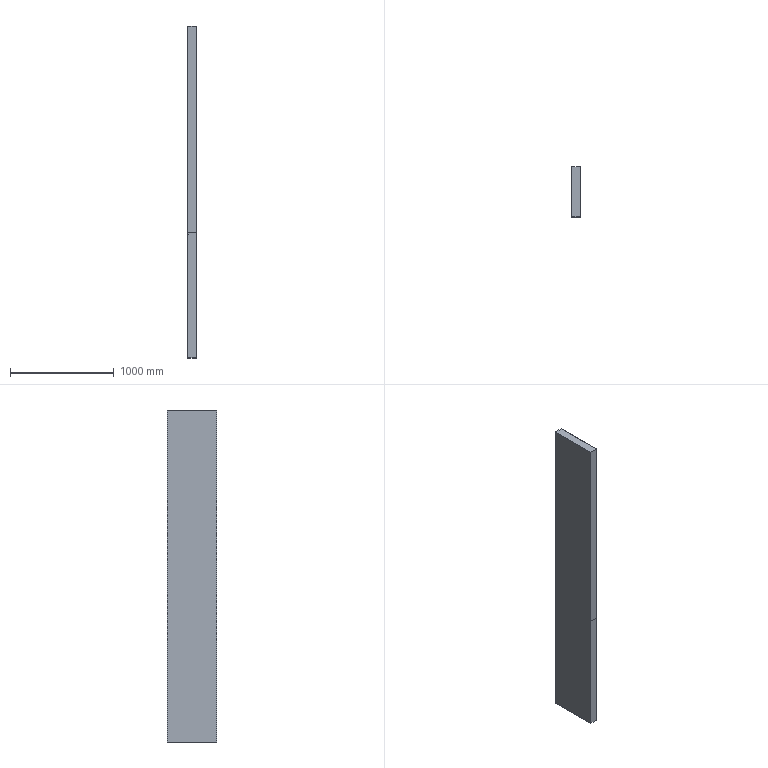Component | NX | CB4_2 | 1 solid | 32 faces | volume 3301326 mm3 | plane 32